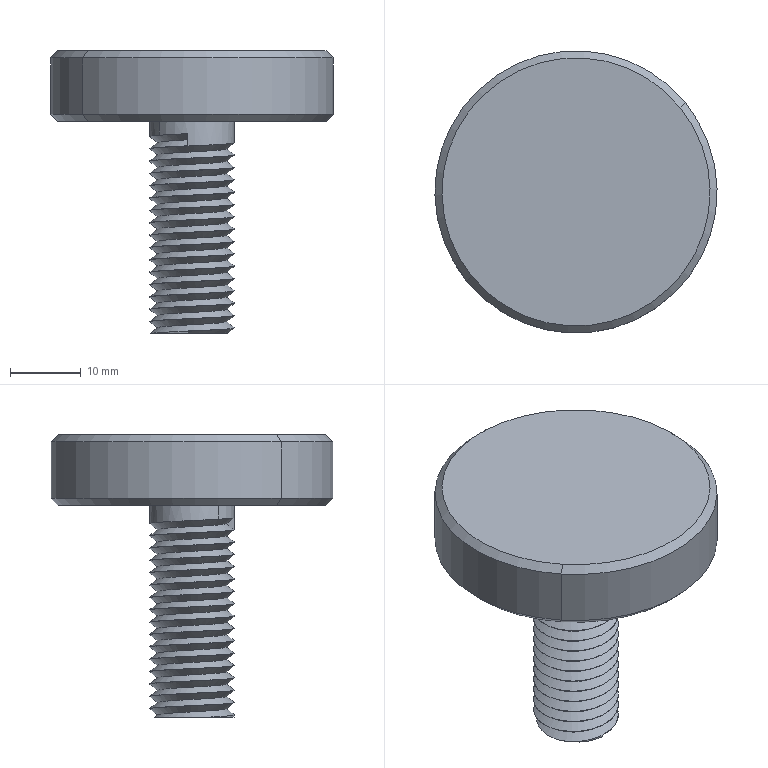Component | SolidWorks | ChassisWheel-2 | 1 solid | 46 faces | volume 15302 mm3 | cylinder 35 | plane 5 | cone 4 | spline 2 | commonest cylinder face diameters 12 x33 40 x2